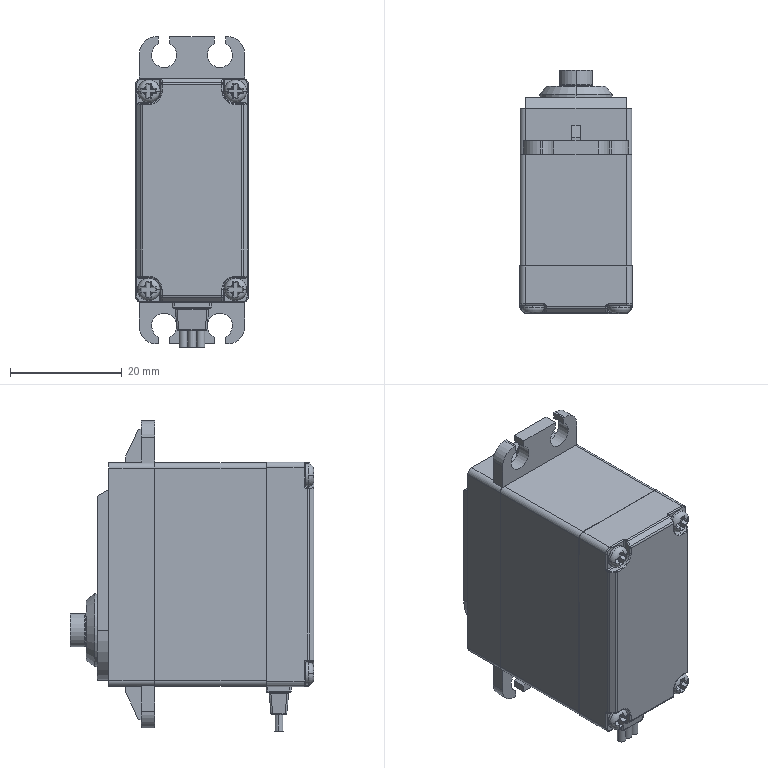Component | SolidWorks | MG996RServo_stp-1 | 11 solids | 454 faces | volume 25965 mm3 | plane 197 | cylinder 163 | spline 78 | torus 12 | cone 4 | commonest cylinder face diameters 0.4 x52 2 x36 1 x16 4 x10 0.6 x8 6 x8 1.5 x6 4.5 x6 | material 45